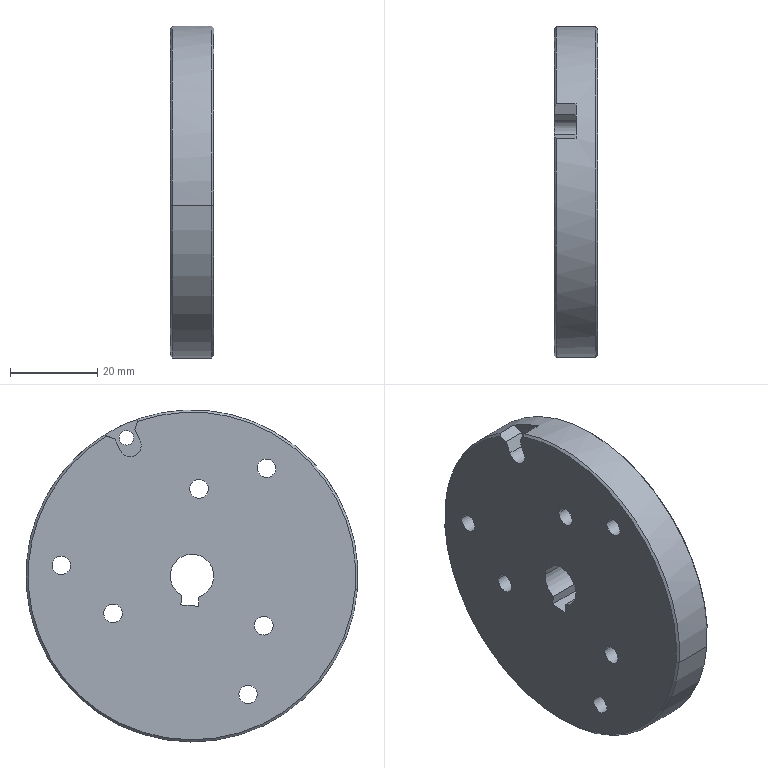Component | SolidWorks | 2018SOLIDWORKS1000000022-1 | 1 solid | 45 faces | volume 42864 mm3 | cylinder 27 | plane 13 | cone 5 | commonest cylinder face diameters 8 x6 4.3 x6 4.2 x6 10 x3 3.3 x2 5 x2 76 x2 | material 6061 Alloy